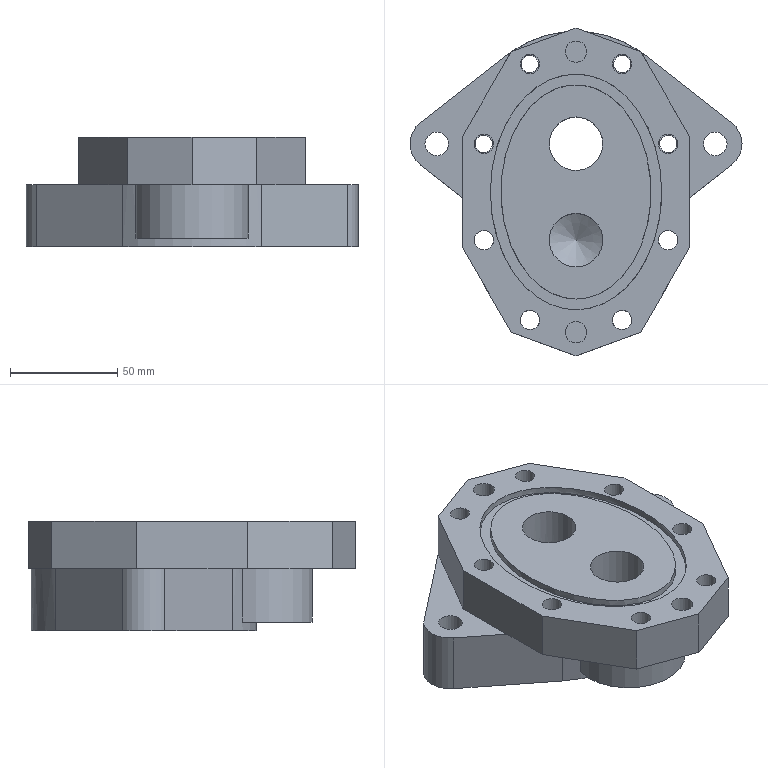Component | NX | CLYB_04_FRONTPUMPCOVER | 1 solid | 86 faces | volume 529681 mm3 | plane 42 | cylinder 35 | cone 7 | other 2 | commonest cylinder face diameters 9 x8 15 x8 25 x4 8 x4 3.3 x3 105 x2 11 x2 10 x2